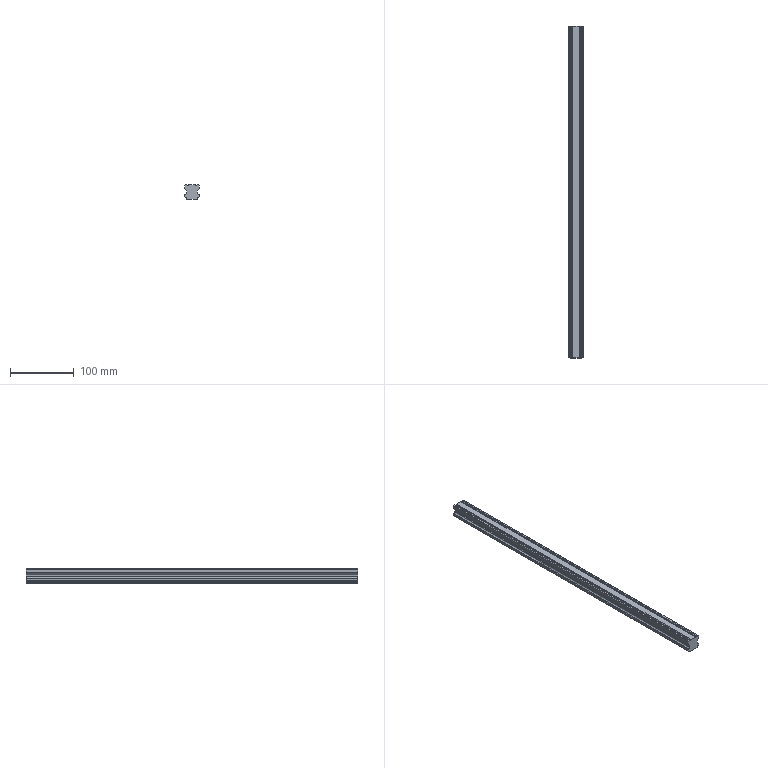Component | SolidWorks | GuideRailHGH25-2-1 | 1 solid | 34 faces | box 23 x 520 x 22 mm | volume 228766 mm3 | plane 30 | cylinder 4 | commonest cylinder face diameters 4.6 x4
build123d program:
from build123d import *

# Parameters (mm, degrees)
BOSS_EXTRUDE1_DEPTH = 260


with BuildPart() as part:
    # Sketch1 → Boss-Extrude1 (new, symmetric)
    with BuildSketch(Plane.XY):
        with BuildLine():
            Line((-10.5, 0), (-8.214, 0))
            Line((-8.214, 0), (-7.448, 0.7667))
            Line((-7.448, 0.7667), (-5.695, 0.7667))
            Line((-5.695, 0.7667), (-4.929, 0))
            Line((-4.929, 0), (4.929, 0))
            Line((4.929, 0), (5.695, 0.7667))
            Line((5.695, 0.7667), (7.448, 0.7667))
            Line((7.448, 0.7667), (8.214, 0))
            Line((8.214, 0), (10.5, 0))
            Line((10.5, 0), (11.5, 1))
            Line((11.5, 1), (11.5, 5.5))
            Line((11.5, 5.5), (8.05, 8.95))
            Line((8.05, 8.95), (8.05, 11.95))
            Line((8.05, 11.95), (8.699, 12.599))
            ThreePointArc((8.699, 12.599), (9.368, 14.082), (10.851, 14.751))
            Line((10.851, 14.751), (11.5, 15.4))
            Line((11.5, 15.4), (11.5, 18.55))
            Line((11.5, 18.55), (10.851, 19.199))
            ThreePointArc((10.851, 19.199), (9.368, 19.868), (8.699, 21.351))
            Line((8.699, 21.351), (8.05, 22))
            Line((8.05, 22), (-8.05, 22))
            Line((-8.05, 22), (-8.699, 21.351))
            ThreePointArc((-8.699, 21.351), (-9.368, 19.868), (-10.851, 19.199))
            Line((-10.851, 19.199), (-11.5, 18.55))
            Line((-11.5, 18.55), (-11.5, 15.4))
            Line((-11.5, 15.4), (-10.851, 14.751))
            ThreePointArc((-10.851, 14.751), (-9.368, 14.082), (-8.699, 12.599))
            Line((-8.699, 12.599), (-8.05, 11.95))
            Line((-8.05, 11.95), (-8.05, 8.95))
            Line((-8.05, 8.95), (-11.5, 5.5))
            Line((-11.5, 5.5), (-11.5, 1))
            Line((-11.5, 1), (-10.5, 0))
        make_face()
    extrude(amount=BOSS_EXTRUDE1_DEPTH, both=True)


solid = part.part

# Placed as in the assembly
solid = solid.moved(Location((90.729, -43.5, -24.5), (-90, 0, 0)))
STEP:
#1=COLOUR_RGB('',0.7922,0.8196,0.9333);
#2=FILL_AREA_STYLE_COLOUR('',#1);
#3=FILL_AREA_STYLE('',(#2));
#4=SURFACE_STYLE_FILL_AREA(#3);
#5=SURFACE_SIDE_STYLE('',(#4));
#6=SURFACE_STYLE_USAGE(.BOTH.,#5);
#7=PRESENTATION_STYLE_ASSIGNMENT((#6));
#8=CARTESIAN_POINT('',(3.915,-11.949,-1.805));
#9=VERTEX_POINT('',#8);
#10=CARTESIAN_POINT('',(3.889,-11.949,-1.831));
#11=VERTEX_POINT('',#10);
#12=CARTESIAN_POINT('',(3.915,-11.949,-1.805));
#13=DIRECTION('',(-0.7071,0.,-0.7071));
#14=VECTOR('',#13,39.37);
#15=LINE('',#12,#14);
#16=EDGE_CURVE('',#9,#11,#15,.T.);
#17=ORIENTED_EDGE('',*,*,#16,.T.);
#18=CARTESIAN_POINT('',(3.889,8.524,-1.831));
#19=VERTEX_POINT('',#18);
#20=CARTESIAN_POINT('',(3.889,8.524,-1.831));
#21=DIRECTION('',(0.,-1.,-0.));
#22=VECTOR('',#21,39.37);
#23=LINE('',#20,#22);
#24=EDGE_CURVE('',#19,#11,#23,.T.);
#25=ORIENTED_EDGE('',*,*,#24,.F.);
#26=CARTESIAN_POINT('',(3.915,8.524,-1.805));
#27=VERTEX_POINT('',#26);
#28=CARTESIAN_POINT('',(3.915,8.524,-1.805));
#29=DIRECTION('',(-0.7071,0.,-0.7071));
#30=VECTOR('',#29,39.37);
#31=LINE('',#28,#30);
#32=EDGE_CURVE('',#27,#19,#31,.T.);
#33=ORIENTED_EDGE('',*,*,#32,.F.);
#34=CARTESIAN_POINT('',(3.915,8.524,-1.805));
#35=DIRECTION('',(0.,-1.,-0.));
#36=VECTOR('',#35,39.37);
#37=LINE('',#34,#36);
#38=EDGE_CURVE('',#27,#9,#37,.T.);
#39=ORIENTED_EDGE('',*,*,#38,.T.);
#40=EDGE_LOOP('',(#17,#25,#33,#39));
#41=FACE_OUTER_BOUND('',#40,.T.);
#42=CARTESIAN_POINT('',(3.915,8.524,-1.805));
#43=DIRECTION('',(-0.7071,-0.,0.7071));
#44=DIRECTION('',(0.7071,-0.,0.7071));
#45=AXIS2_PLACEMENT_3D('',#42,#43,#44);
#46=PLANE('',#45);
#47=ADVANCED_FACE('',(#41),#46,.F.);
#48=CARTESIAN_POINT('',(3.255,-11.949,-1.831));
#49=VERTEX_POINT('',#48);
#50=CARTESIAN_POINT('',(3.889,-11.949,-1.831));
#51=DIRECTION('',(-1.,-0.,-0.));
#52=VECTOR('',#51,39.37);
#53=LINE('',#50,#52);
#54=EDGE_CURVE('',#11,#49,#53,.T.);
#55=ORIENTED_EDGE('',*,*,#54,.T.);
#56=CARTESIAN_POINT('',(3.255,8.524,-1.831));
#57=VERTEX_POINT('',#56);
#58=CARTESIAN_POINT('',(3.255,8.524,-1.831));
#59=DIRECTION('',(0.,-1.,-0.));
#60=VECTOR('',#59,39.37);
#61=LINE('',#58,#60);
#62=EDGE_CURVE('',#57,#49,#61,.T.);
#63=ORIENTED_EDGE('',*,*,#62,.F.);
#64=CARTESIAN_POINT('',(3.889,8.524,-1.831));
#65=DIRECTION('',(-1.,-0.,-0.));
#66=VECTOR('',#65,39.37);
#67=LINE('',#64,#66);
#68=EDGE_CURVE('',#19,#57,#67,.T.);
#69=ORIENTED_EDGE('',*,*,#68,.F.);
#70=ORIENTED_EDGE('',*,*,#24,.T.);
#71=EDGE_LOOP('',(#55,#63,#69,#70));
#72=FACE_OUTER_BOUND('',#71,.T.);
#73=CARTESIAN_POINT('',(3.889,8.524,-1.831));
#74=DIRECTION('',(-0.,-0.,1.));
#75=DIRECTION('',(1.,0.,0.));
#76=AXIS2_PLACEMENT_3D('',#73,#74,#75);
#77=PLANE('',#76);
#78=ADVANCED_FACE('',(#72),#77,.F.);
#79=CARTESIAN_POINT('',(3.23,-11.949,-1.805));
#80=VERTEX_POINT('',#79);
#81=CARTESIAN_POINT('',(3.255,-11.949,-1.831));
#82=DIRECTION('',(-0.7071,-0.,0.7071));
#83=VECTOR('',#82,39.37);
#84=LINE('',#81,#83);
#85=EDGE_CURVE('',#49,#80,#84,.T.);
#86=ORIENTED_EDGE('',*,*,#85,.T.);
#87=CARTESIAN_POINT('',(3.23,8.524,-1.805));
#88=VERTEX_POINT('',#87);
#89=CARTESIAN_POINT('',(3.23,8.524,-1.805));
#90=DIRECTION('',(0.,-1.,-0.));
#91=VECTOR('',#90,39.37);
#92=LINE('',#89,#91);
#93=EDGE_CURVE('',#88,#80,#92,.T.);
#94=ORIENTED_EDGE('',*,*,#93,.F.);
#95=CARTESIAN_POINT('',(3.255,8.524,-1.831));
#96=DIRECTION('',(-0.7071,-0.,0.7071));
#97=VECTOR('',#96,39.37);
#98=LINE('',#95,#97);
#99=EDGE_CURVE('',#57,#88,#98,.T.);
#100=ORIENTED_EDGE('',*,*,#99,.F.);
#101=ORIENTED_EDGE('',*,*,#62,.T.);
#102=EDGE_LOOP('',(#86,#94,#100,#101));
#103=FACE_OUTER_BOUND('',#102,.T.);
#104=CARTESIAN_POINT('',(3.255,8.524,-1.831));
#105=DIRECTION('',(0.7071,-0.,0.7071));
#106=DIRECTION('',(0.7071,0.,-0.7071));
#107=AXIS2_PLACEMENT_3D('',#104,#105,#106);
#108=PLANE('',#107);
#109=ADVANCED_FACE('',(#103),#108,.F.);
#110=CARTESIAN_POINT('',(3.145,-11.949,-1.72));
#111=VERTEX_POINT('',#110);
#112=CARTESIAN_POINT('',(3.139,-11.949,-1.811));
#113=DIRECTION('',(-0.,1.,0.));
#114=DIRECTION('',(1.,0.,0.));
#115=AXIS2_PLACEMENT_3D('',#112,#113,#114);
#116=CIRCLE('',#115,0.09055);
#117=EDGE_CURVE('',#111,#80,#116,.T.);
#118=ORIENTED_EDGE('',*,*,#117,.F.);
#119=CARTESIAN_POINT('',(3.145,8.524,-1.72));
#120=VERTEX_POINT('',#119);
#121=CARTESIAN_POINT('',(3.145,8.524,-1.72));
#122=DIRECTION('',(0.,-1.,-0.));
#123=VECTOR('',#122,39.37);
#124=LINE('',#121,#123);
#125=EDGE_CURVE('',#120,#111,#124,.T.);
#126=ORIENTED_EDGE('',*,*,#125,.F.);
#127=CARTESIAN_POINT('',(3.139,8.524,-1.811));
#128=DIRECTION('',(-0.,1.,0.));
#129=DIRECTION('',(1.,0.,0.));
#130=AXIS2_PLACEMENT_3D('',#127,#128,#129);
#131=CIRCLE('',#130,0.09055);
#132=EDGE_CURVE('',#120,#88,#131,.T.);
#133=ORIENTED_EDGE('',*,*,#132,.T.);
#134=ORIENTED_EDGE('',*,*,#93,.T.);
#135=EDGE_LOOP('',(#118,#126,#133,#134));
#136=FACE_OUTER_BOUND('',#135,.T.);
#137=CARTESIAN_POINT('',(3.139,8.524,-1.811));
#138=DIRECTION('',(0.,-1.,-0.));
#139=DIRECTION('',(-1.,0.,-0.));
#140=AXIS2_PLACEMENT_3D('',#137,#138,#139);
#141=CYLINDRICAL_SURFACE('',#140,0.09055);
#142=ADVANCED_FACE('',(#136),#141,.F.);
#143=CARTESIAN_POINT('',(3.119,-11.949,-1.695));
#144=VERTEX_POINT('',#143);
#145=CARTESIAN_POINT('',(3.145,-11.949,-1.72));
#146=DIRECTION('',(-0.7071,-0.,0.7071));
#147=VECTOR('',#146,39.37);
#148=LINE('',#145,#147);
#149=EDGE_CURVE('',#111,#144,#148,.T.);
#150=ORIENTED_EDGE('',*,*,#149,.T.);
#151=CARTESIAN_POINT('',(3.119,8.524,-1.695));
#152=VERTEX_POINT('',#151);
#153=CARTESIAN_POINT('',(3.119,8.524,-1.695));
#154=DIRECTION('',(0.,-1.,-0.));
#155=VECTOR('',#154,39.37);
#156=LINE('',#153,#155);
#157=EDGE_CURVE('',#152,#144,#156,.T.);
#158=ORIENTED_EDGE('',*,*,#157,.F.);
#159=CARTESIAN_POINT('',(3.145,8.524,-1.72));
#160=DIRECTION('',(-0.7071,-0.,0.7071));
#161=VECTOR('',#160,39.37);
#162=LINE('',#159,#161);
#163=EDGE_CURVE('',#120,#152,#162,.T.);
#164=ORIENTED_EDGE('',*,*,#163,.F.);
#165=ORIENTED_EDGE('',*,*,#125,.T.);
#166=EDGE_LOOP('',(#150,#158,#164,#165));
#167=FACE_OUTER_BOUND('',#166,.T.);
#168=CARTESIAN_POINT('',(3.145,8.524,-1.72));
#169=DIRECTION('',(0.7071,-0.,0.7071));
#170=DIRECTION('',(0.7071,0.,-0.7071));
#171=AXIS2_PLACEMENT_3D('',#168,#169,#170);
#172=PLANE('',#171);
#173=ADVANCED_FACE('',(#167),#172,.F.);
#174=CARTESIAN_POINT('',(3.119,-11.949,-1.571));
#175=VERTEX_POINT('',#174);
#176=CARTESIAN_POINT('',(3.119,-11.949,-1.695));
#177=DIRECTION('',(-0.,-0.,1.));
#178=VECTOR('',#177,39.37);
#179=LINE('',#176,#178);
#180=EDGE_CURVE('',#144,#175,#179,.T.);
#181=ORIENTED_EDGE('',*,*,#180,.T.);
#182=CARTESIAN_POINT('',(3.119,8.524,-1.571));
#183=VERTEX_POINT('',#182);
#184=CARTESIAN_POINT('',(3.119,8.524,-1.571));
#185=DIRECTION('',(0.,-1.,-0.));
#186=VECTOR('',#185,39.37);
#187=LINE('',#184,#186);
#188=EDGE_CURVE('',#183,#175,#187,.T.);
#189=ORIENTED_EDGE('',*,*,#188,.F.);
#190=CARTESIAN_POINT('',(3.119,8.524,-1.695));
#191=DIRECTION('',(-0.,-0.,1.));
#192=VECTOR('',#191,39.37);
#193=LINE('',#190,#192);
#194=EDGE_CURVE('',#152,#183,#193,.T.);
#195=ORIENTED_EDGE('',*,*,#194,.F.);
#196=ORIENTED_EDGE('',*,*,#157,.T.);
#197=EDGE_LOOP('',(#181,#189,#195,#196));
#198=FACE_OUTER_BOUND('',#197,.T.);
#199=CARTESIAN_POINT('',(3.119,8.524,-1.695));
#200=DIRECTION('',(1.,0.,0.));
#201=DIRECTION('',(0.,-1.,-0.));
#202=AXIS2_PLACEMENT_3D('',#199,#200,#201);
#203=PLANE('',#202);
#204=ADVANCED_FACE('',(#198),#203,.F.);
#205=CARTESIAN_POINT('',(3.145,-11.949,-1.545));
#206=VERTEX_POINT('',#205);
#207=CARTESIAN_POINT('',(3.119,-11.949,-1.571));
#208=DIRECTION('',(0.7071,-0.,0.7071));
#209=VECTOR('',#208,39.37);
#210=LINE('',#207,#209);
#211=EDGE_CURVE('',#175,#206,#210,.T.);
#212=ORIENTED_EDGE('',*,*,#211,.T.);
#213=CARTESIAN_POINT('',(3.145,8.524,-1.545));
#214=VERTEX_POINT('',#213);
#215=CARTESIAN_POINT('',(3.145,8.524,-1.545));
#216=DIRECTION('',(0.,-1.,-0.));
#217=VECTOR('',#216,39.37);
#218=LINE('',#215,#217);
#219=EDGE_CURVE('',#214,#206,#218,.T.);
#220=ORIENTED_EDGE('',*,*,#219,.F.);
#221=CARTESIAN_POINT('',(3.119,8.524,-1.571));
#222=DIRECTION('',(0.7071,-0.,0.7071));
#223=VECTOR('',#222,39.37);
#224=LINE('',#221,#223);
#225=EDGE_CURVE('',#183,#214,#224,.T.);
#226=ORIENTED_EDGE('',*,*,#225,.F.);
#227=ORIENTED_EDGE('',*,*,#188,.T.);
#228=EDGE_LOOP('',(#212,#220,#226,#227));
#229=FACE_OUTER_BOUND('',#228,.T.);
#230=CARTESIAN_POINT('',(3.119,8.524,-1.571));
#231=DIRECTION('',(0.7071,0.,-0.7071));
#232=DIRECTION('',(-0.7071,0.,-0.7071));
#233=AXIS2_PLACEMENT_3D('',#230,#231,#232);
#234=PLANE('',#233);
#235=ADVANCED_FACE('',(#229),#234,.F.);
#236=CARTESIAN_POINT('',(3.23,-11.949,-1.461));
#237=VERTEX_POINT('',#236);
#238=CARTESIAN_POINT('',(3.139,-11.949,-1.455));
#239=DIRECTION('',(-0.,1.,0.));
#240=DIRECTION('',(1.,0.,0.));
#241=AXIS2_PLACEMENT_3D('',#238,#239,#240);
#242=CIRCLE('',#241,0.09055);
#243=EDGE_CURVE('',#237,#206,#242,.T.);
#244=ORIENTED_EDGE('',*,*,#243,.F.);
#245=CARTESIAN_POINT('',(3.23,8.524,-1.461));
#246=VERTEX_POINT('',#245);
#247=CARTESIAN_POINT('',(3.23,8.524,-1.461));
#248=DIRECTION('',(0.,-1.,-0.));
#249=VECTOR('',#248,39.37);
#250=LINE('',#247,#249);
#251=EDGE_CURVE('',#246,#237,#250,.T.);
#252=ORIENTED_EDGE('',*,*,#251,.F.);
#253=CARTESIAN_POINT('',(3.139,8.524,-1.455));
#254=DIRECTION('',(-0.,1.,0.));
#255=DIRECTION('',(1.,0.,0.));
#256=AXIS2_PLACEMENT_3D('',#253,#254,#255);
#257=CIRCLE('',#256,0.09055);
#258=EDGE_CURVE('',#246,#214,#257,.T.);
#259=ORIENTED_EDGE('',*,*,#258,.T.);
#260=ORIENTED_EDGE('',*,*,#219,.T.);
#261=EDGE_LOOP('',(#244,#252,#259,#260));
#262=FACE_OUTER_BOUND('',#261,.T.);
#263=CARTESIAN_POINT('',(3.139,8.524,-1.455));
#264=DIRECTION('',(0.,-1.,-0.));
#265=DIRECTION('',(-1.,0.,-0.));
#266=AXIS2_PLACEMENT_3D('',#263,#264,#265);
#267=CYLINDRICAL_SURFACE('',#266,0.09055);
#268=ADVANCED_FACE('',(#262),#267,.F.);
#269=CARTESIAN_POINT('',(3.255,-11.949,-1.435));
#270=VERTEX_POINT('',#269);
#271=CARTESIAN_POINT('',(3.23,-11.949,-1.461));
#272=DIRECTION('',(0.7071,-0.,0.7071));
#273=VECTOR('',#272,39.37);
#274=LINE('',#271,#273);
#275=EDGE_CURVE('',#237,#270,#274,.T.);
#276=ORIENTED_EDGE('',*,*,#275,.T.);
#277=CARTESIAN_POINT('',(3.255,8.524,-1.435));
#278=VERTEX_POINT('',#277);
#279=CARTESIAN_POINT('',(3.255,8.524,-1.435));
#280=DIRECTION('',(0.,-1.,-0.));
#281=VECTOR('',#280,39.37);
#282=LINE('',#279,#281);
#283=EDGE_CURVE('',#278,#270,#282,.T.);
#284=ORIENTED_EDGE('',*,*,#283,.F.);
#285=CARTESIAN_POINT('',(3.23,8.524,-1.461));
#286=DIRECTION('',(0.7071,-0.,0.7071));
#287=VECTOR('',#286,39.37);
#288=LINE('',#285,#287);
#289=EDGE_CURVE('',#246,#278,#288,.T.);
#290=ORIENTED_EDGE('',*,*,#289,.F.);
#291=ORIENTED_EDGE('',*,*,#251,.T.);
#292=EDGE_LOOP('',(#276,#284,#290,#291));
#293=FACE_OUTER_BOUND('',#292,.T.);
#294=CARTESIAN_POINT('',(3.23,8.524,-1.461));
#295=DIRECTION('',(0.7071,0.,-0.7071));
#296=DIRECTION('',(-0.7071,0.,-0.7071));
#297=AXIS2_PLACEMENT_3D('',#294,#295,#296);
#298=PLANE('',#297);
#299=ADVANCED_FACE('',(#293),#298,.F.);
#300=CARTESIAN_POINT('',(3.255,-11.949,-1.317));
#301=VERTEX_POINT('',#300);
#302=CARTESIAN_POINT('',(3.255,-11.949,-1.435));
#303=DIRECTION('',(-0.,-0.,1.));
#304=VECTOR('',#303,39.37);
#305=LINE('',#302,#304);
#306=EDGE_CURVE('',#270,#301,#305,.T.);
#307=ORIENTED_EDGE('',*,*,#306,.T.);
#308=CARTESIAN_POINT('',(3.255,8.524,-1.317));
#309=VERTEX_POINT('',#308);
#310=CARTESIAN_POINT('',(3.255,8.524,-1.317));
#311=DIRECTION('',(0.,-1.,-0.));
#312=VECTOR('',#311,39.37);
#313=LINE('',#310,#312);
#314=EDGE_CURVE('',#309,#301,#313,.T.);
#315=ORIENTED_EDGE('',*,*,#314,.F.);
#316=CARTESIAN_POINT('',(3.255,8.524,-1.435));
#317=DIRECTION('',(-0.,-0.,1.));
#318=VECTOR('',#317,39.37);
#319=LINE('',#316,#318);
#320=EDGE_CURVE('',#278,#309,#319,.T.);
#321=ORIENTED_EDGE('',*,*,#320,.F.);
#322=ORIENTED_EDGE('',*,*,#283,.T.);
#323=EDGE_LOOP('',(#307,#315,#321,#322));
#324=FACE_OUTER_BOUND('',#323,.T.);
#325=CARTESIAN_POINT('',(3.255,8.524,-1.435));
#326=DIRECTION('',(1.,0.,0.));
#327=DIRECTION('',(0.,0.,-1.));
#328=AXIS2_PLACEMENT_3D('',#325,#326,#327);
#329=PLANE('',#328);
#330=ADVANCED_FACE('',(#324),#329,.F.);
#331=CARTESIAN_POINT('',(3.119,-11.949,-1.181));
#332=VERTEX_POINT('',#331);
#333=CARTESIAN_POINT('',(3.255,-11.949,-1.317));
#334=DIRECTION('',(-0.7071,-0.,0.7071));
#335=VECTOR('',#334,39.37);
#336=LINE('',#333,#335);
#337=EDGE_CURVE('',#301,#332,#336,.T.);
#338=ORIENTED_EDGE('',*,*,#337,.T.);
#339=CARTESIAN_POINT('',(3.119,8.524,-1.181));
#340=VERTEX_POINT('',#339);
#341=CARTESIAN_POINT('',(3.119,8.524,-1.181));
#342=DIRECTION('',(0.,-1.,-0.));
#343=VECTOR('',#342,39.37);
#344=LINE('',#341,#343);
#345=EDGE_CURVE('',#340,#332,#344,.T.);
#346=ORIENTED_EDGE('',*,*,#345,.F.);
#347=CARTESIAN_POINT('',(3.255,8.524,-1.317));
#348=DIRECTION('',(-0.7071,-0.,0.7071));
#349=VECTOR('',#348,39.37);
#350=LINE('',#347,#349);
#351=EDGE_CURVE('',#309,#340,#350,.T.);
#352=ORIENTED_EDGE('',*,*,#351,.F.);
#353=ORIENTED_EDGE('',*,*,#314,.T.);
#354=EDGE_LOOP('',(#338,#346,#352,#353));
#355=FACE_OUTER_BOUND('',#354,.T.);
#356=CARTESIAN_POINT('',(3.255,8.524,-1.317));
#357=DIRECTION('',(0.7071,-0.,0.7071));
#358=DIRECTION('',(0.7071,0.,-0.7071));
#359=AXIS2_PLACEMENT_3D('',#356,#357,#358);
#360=PLANE('',#359);
#361=ADVANCED_FACE('',(#355),#360,.F.);
#362=CARTESIAN_POINT('',(3.119,-11.949,-1.004));
#363=VERTEX_POINT('',#362);
#364=CARTESIAN_POINT('',(3.119,-11.949,-1.181));
#365=DIRECTION('',(-0.,-0.,1.));
#366=VECTOR('',#365,39.37);
#367=LINE('',#364,#366);
#368=EDGE_CURVE('',#332,#363,#367,.T.);
#369=ORIENTED_EDGE('',*,*,#368,.T.);
#370=CARTESIAN_POINT('',(3.119,8.524,-1.004));
#371=VERTEX_POINT('',#370);
#372=CARTESIAN_POINT('',(3.119,8.524,-1.004));
#373=DIRECTION('',(0.,-1.,-0.));
#374=VECTOR('',#373,39.37);
#375=LINE('',#372,#374);
#376=EDGE_CURVE('',#371,#363,#375,.T.);
#377=ORIENTED_EDGE('',*,*,#376,.F.);
#378=CARTESIAN_POINT('',(3.119,8.524,-1.181));
#379=DIRECTION('',(-0.,-0.,1.));
#380=VECTOR('',#379,39.37);
#381=LINE('',#378,#380);
#382=EDGE_CURVE('',#340,#371,#381,.T.);
#383=ORIENTED_EDGE('',*,*,#382,.F.);
#384=ORIENTED_EDGE('',*,*,#345,.T.);
#385=EDGE_LOOP('',(#369,#377,#383,#384));
#386=FACE_OUTER_BOUND('',#385,.T.);
#387=CARTESIAN_POINT('',(3.119,8.524,-1.181));
#388=DIRECTION('',(1.,0.,0.));
#389=DIRECTION('',(0.,-1.,-0.));
#390=AXIS2_PLACEMENT_3D('',#387,#388,#389);
#391=PLANE('',#390);
#392=ADVANCED_FACE('',(#386),#391,.F.);
#393=CARTESIAN_POINT('',(3.159,-11.949,-0.9646));
#394=VERTEX_POINT('',#393);
#395=CARTESIAN_POINT('',(3.119,-11.949,-1.004));
#396=DIRECTION('',(0.7071,-0.,0.7071));
#397=VECTOR('',#396,39.37);
#398=LINE('',#395,#397);
#399=EDGE_CURVE('',#363,#394,#398,.T.);
#400=ORIENTED_EDGE('',*,*,#399,.T.);
#401=CARTESIAN_POINT('',(3.159,8.524,-0.9646));
#402=VERTEX_POINT('',#401);
#403=CARTESIAN_POINT('',(3.159,8.524,-0.9646));
#404=DIRECTION('',(0.,-1.,-0.));
#405=VECTOR('',#404,39.37);
#406=LINE('',#403,#405);
#407=EDGE_CURVE('',#402,#394,#406,.T.);
#408=ORIENTED_EDGE('',*,*,#407,.F.);
#409=CARTESIAN_POINT('',(3.119,8.524,-1.004));
#410=DIRECTION('',(0.7071,-0.,0.7071));
#411=VECTOR('',#410,39.37);
#412=LINE('',#409,#411);
#413=EDGE_CURVE('',#371,#402,#412,.T.);
#414=ORIENTED_EDGE('',*,*,#413,.F.);
#415=ORIENTED_EDGE('',*,*,#376,.T.);
#416=EDGE_LOOP('',(#400,#408,#414,#415));
#417=FACE_OUTER_BOUND('',#416,.T.);
#418=CARTESIAN_POINT('',(3.119,8.524,-1.004));
#419=DIRECTION('',(0.7071,0.,-0.7071));
#420=DIRECTION('',(-0.7071,0.,-0.7071));
#421=AXIS2_PLACEMENT_3D('',#418,#419,#420);
#422=PLANE('',#421);
#423=ADVANCED_FACE('',(#417),#422,.F.);
#424=CARTESIAN_POINT('',(3.249,-11.949,-0.9646));
#425=VERTEX_POINT('',#424);
#426=CARTESIAN_POINT('',(3.159,-11.949,-0.9646));
#427=DIRECTION('',(1.,0.,0.));
#428=VECTOR('',#427,39.37);
#429=LINE('',#426,#428);
#430=EDGE_CURVE('',#394,#425,#429,.T.);
#431=ORIENTED_EDGE('',*,*,#430,.T.);
#432=CARTESIAN_POINT('',(3.249,8.524,-0.9646));
#433=VERTEX_POINT('',#432);
#434=CARTESIAN_POINT('',(3.249,8.524,-0.9646));
#435=DIRECTION('',(0.,-1.,-0.));
#436=VECTOR('',#435,39.37);
#437=LINE('',#434,#436);
#438=EDGE_CURVE('',#433,#425,#437,.T.);
#439=ORIENTED_EDGE('',*,*,#438,.F.);
#440=CARTESIAN_POINT('',(3.159,8.524,-0.9646));
#441=DIRECTION('',(1.,0.,0.));
#442=VECTOR('',#441,39.37);
#443=LINE('',#440,#442);
#444=EDGE_CURVE('',#402,#433,#443,.T.);
#445=ORIENTED_EDGE('',*,*,#444,.F.);
#446=ORIENTED_EDGE('',*,*,#407,.T.);
#447=EDGE_LOOP('',(#431,#439,#445,#446));
#448=FACE_OUTER_BOUND('',#447,.T.);
#449=CARTESIAN_POINT('',(3.159,8.524,-0.9646));
#450=DIRECTION('',(0.,0.,-1.));
#451=DIRECTION('',(-1.,-0.,-0.));
#452=AXIS2_PLACEMENT_3D('',#449,#450,#451);
#453=PLANE('',#452);
#454=ADVANCED_FACE('',(#448),#453,.F.);
#455=CARTESIAN_POINT('',(3.279,-11.949,-0.9948));
#456=VERTEX_POINT('',#455);
#457=CARTESIAN_POINT('',(3.249,-11.949,-0.9646));
#458=DIRECTION('',(0.7071,0.,-0.7071));
#459=VECTOR('',#458,39.37);
#460=LINE('',#457,#459);
#461=EDGE_CURVE('',#425,#456,#460,.T.);
#462=ORIENTED_EDGE('',*,*,#461,.T.);
#463=CARTESIAN_POINT('',(3.279,8.524,-0.9948));
#464=VERTEX_POINT('',#463);
#465=CARTESIAN_POINT('',(3.279,8.524,-0.9948));
#466=DIRECTION('',(0.,-1.,-0.));
#467=VECTOR('',#466,39.37);
#468=LINE('',#465,#467);
#469=EDGE_CURVE('',#464,#456,#468,.T.);
#470=ORIENTED_EDGE('',*,*,#469,.F.);
#471=CARTESIAN_POINT('',(3.249,8.524,-0.9646));
#472=DIRECTION('',(0.7071,0.,-0.7071));
#473=VECTOR('',#472,39.37);
#474=LINE('',#471,#473);
#475=EDGE_CURVE('',#433,#464,#474,.T.);
#476=ORIENTED_EDGE('',*,*,#475,.F.);
#477=ORIENTED_EDGE('',*,*,#438,.T.);
#478=EDGE_LOOP('',(#462,#470,#476,#477));
#479=FACE_OUTER_BOUND('',#478,.T.);
#480=CARTESIAN_POINT('',(3.249,8.524,-0.9646));
#481=DIRECTION('',(-0.7071,0.,-0.7071));
#482=DIRECTION('',(-0.7071,-0.,0.7071));
#483=AXIS2_PLACEMENT_3D('',#480,#481,#482);
#484=PLANE('',#483);
#485=ADVANCED_FACE('',(#479),#484,.F.);
#486=CARTESIAN_POINT('',(3.348,-11.949,-0.9948));
#487=VERTEX_POINT('',#486);
#488=CARTESIAN_POINT('',(3.279,-11.949,-0.9948));
#489=DIRECTION('',(1.,0.,-0.));
#490=VECTOR('',#489,39.37);
#491=LINE('',#488,#490);
#492=EDGE_CURVE('',#456,#487,#491,.T.);
#493=ORIENTED_EDGE('',*,*,#492,.T.);
#494=CARTESIAN_POINT('',(3.348,8.524,-0.9948));
#495=VERTEX_POINT('',#494);
#496=CARTESIAN_POINT('',(3.348,8.524,-0.9948));
#497=DIRECTION('',(0.,-1.,-0.));
#498=VECTOR('',#497,39.37);
#499=LINE('',#496,#498);
#500=EDGE_CURVE('',#495,#487,#499,.T.);
#501=ORIENTED_EDGE('',*,*,#500,.F.);
#502=CARTESIAN_POINT('',(3.279,8.524,-0.9948));
#503=DIRECTION('',(1.,0.,-0.));
#504=VECTOR('',#503,39.37);
#505=LINE('',#502,#504);
#506=EDGE_CURVE('',#464,#495,#505,.T.);
#507=ORIENTED_EDGE('',*,*,#506,.F.);
#508=ORIENTED_EDGE('',*,*,#469,.T.);
#509=EDGE_LOOP('',(#493,#501,#507,#508));
#510=FACE_OUTER_BOUND('',#509,.T.);
#511=CARTESIAN_POINT('',(3.279,8.524,-0.9948));
#512=DIRECTION('',(-0.,0.,-1.));
#513=DIRECTION('',(-1.,-0.,0.));
#514=AXIS2_PLACEMENT_3D('',#511,#512,#513);
#515=PLANE('',#514);
#516=ADVANCED_FACE('',(#510),#515,.F.);
#517=CARTESIAN_POINT('',(3.378,-11.949,-0.9646));
#518=VERTEX_POINT('',#517);
#519=CARTESIAN_POINT('',(3.348,-11.949,-0.9948));
#520=DIRECTION('',(0.7071,-0.,0.7071));
#521=VECTOR('',#520,39.37);
#522=LINE('',#519,#521);
#523=EDGE_CURVE('',#487,#518,#522,.T.);
#524=ORIENTED_EDGE('',*,*,#523,.T.);
#525=CARTESIAN_POINT('',(3.378,8.524,-0.9646));
#526=VERTEX_POINT('',#525);
#527=CARTESIAN_POINT('',(3.378,8.524,-0.9646));
#528=DIRECTION('',(0.,-1.,-0.));
#529=VECTOR('',#528,39.37);
#530=LINE('',#527,#529);
#531=EDGE_CURVE('',#526,#518,#530,.T.);
#532=ORIENTED_EDGE('',*,*,#531,.F.);
#533=CARTESIAN_POINT('',(3.348,8.524,-0.9948));
#534=DIRECTION('',(0.7071,-0.,0.7071));
#535=VECTOR('',#534,39.37);
#536=LINE('',#533,#535);
#537=EDGE_CURVE('',#495,#526,#536,.T.);
#538=ORIENTED_EDGE('',*,*,#537,.F.);
#539=ORIENTED_EDGE('',*,*,#500,.T.);
#540=EDGE_LOOP('',(#524,#532,#538,#539));
#541=FACE_OUTER_BOUND('',#540,.T.);
#542=CARTESIAN_POINT('',(3.348,8.524,-0.9948));
#543=DIRECTION('',(0.7071,0.,-0.7071));
#544=DIRECTION('',(-0.7071,0.,-0.7071));
#545=AXIS2_PLACEMENT_3D('',#542,#543,#544);
#546=PLANE('',#545);
#547=ADVANCED_FACE('',(#541),#546,.F.);
#548=CARTESIAN_POINT('',(3.766,-11.949,-0.9646));
#549=VERTEX_POINT('',#548);
#550=CARTESIAN_POINT('',(3.378,-11.949,-0.9646));
#551=DIRECTION('',(1.,0.,0.));
#552=VECTOR('',#551,39.37);
#553=LINE('',#550,#552);
#554=EDGE_CURVE('',#518,#549,#553,.T.);
#555=ORIENTED_EDGE('',*,*,#554,.T.);
#556=CARTESIAN_POINT('',(3.766,8.524,-0.9646));
#557=VERTEX_POINT('',#556);
#558=CARTESIAN_POINT('',(3.766,8.524,-0.9646));
#559=DIRECTION('',(0.,-1.,-0.));
#560=VECTOR('',#559,39.37);
#561=LINE('',#558,#560);
#562=EDGE_CURVE('',#557,#549,#561,.T.);
#563=ORIENTED_EDGE('',*,*,#562,.F.);
#564=CARTESIAN_POINT('',(3.378,8.524,-0.9646));
#565=DIRECTION('',(1.,0.,0.));
#566=VECTOR('',#565,39.37);
#567=LINE('',#564,#566);
#568=EDGE_CURVE('',#526,#557,#567,.T.);
#569=ORIENTED_EDGE('',*,*,#568,.F.);
#570=ORIENTED_EDGE('',*,*,#531,.T.);
#571=EDGE_LOOP('',(#555,#563,#569,#570));
#572=FACE_OUTER_BOUND('',#571,.T.);
#573=CARTESIAN_POINT('',(3.378,8.524,-0.9646));
#574=DIRECTION('',(0.,0.,-1.));
#575=DIRECTION('',(-1.,-0.,-0.));
#576=AXIS2_PLACEMENT_3D('',#573,#574,#575);
#577=PLANE('',#576);
#578=ADVANCED_FACE('',(#572),#577,.F.);
#579=CARTESIAN_POINT('',(3.796,-11.949,-0.9948));
#580=VERTEX_POINT('',#579);
#581=CARTESIAN_POINT('',(3.766,-11.949,-0.9646));
#582=DIRECTION('',(0.7071,0.,-0.7071));
#583=VECTOR('',#582,39.37);
#584=LINE('',#581,#583);
#585=EDGE_CURVE('',#549,#580,#584,.T.);
#586=ORIENTED_EDGE('',*,*,#585,.T.);
#587=CARTESIAN_POINT('',(3.796,8.524,-0.9948));
#588=VERTEX_POINT('',#587);
#589=CARTESIAN_POINT('',(3.796,8.524,-0.9948));
#590=DIRECTION('',(0.,-1.,-0.));
#591=VECTOR('',#590,39.37);
#592=LINE('',#589,#591);
#593=EDGE_CURVE('',#588,#580,#592,.T.);
#594=ORIENTED_EDGE('',*,*,#593,.F.);
#595=CARTESIAN_POINT('',(3.766,8.524,-0.9646));
#596=DIRECTION('',(0.7071,0.,-0.7071));
#597=VECTOR('',#596,39.37);
#598=LINE('',#595,#597);
#599=EDGE_CURVE('',#557,#588,#598,.T.);
#600=ORIENTED_EDGE('',*,*,#599,.F.);
#601=ORIENTED_EDGE('',*,*,#562,.T.);
#602=EDGE_LOOP('',(#586,#594,#600,#601));
#603=FACE_OUTER_BOUND('',#602,.T.);
#604=CARTESIAN_POINT('',(3.766,8.524,-0.9646));
#605=DIRECTION('',(-0.7071,0.,-0.7071));
#606=DIRECTION('',(-0.7071,-0.,0.7071));
#607=AXIS2_PLACEMENT_3D('',#604,#605,#606);
#608=PLANE('',#607);
#609=ADVANCED_FACE('',(#603),#608,.F.);
#610=CARTESIAN_POINT('',(3.865,-11.949,-0.9948));
#611=VERTEX_POINT('',#610);
#612=CARTESIAN_POINT('',(3.796,-11.949,-0.9948));
#613=DIRECTION('',(1.,0.,0.));
#614=VECTOR('',#613,39.37);
#615=LINE('',#612,#614);
#616=EDGE_CURVE('',#580,#611,#615,.T.);
#617=ORIENTED_EDGE('',*,*,#616,.T.);
#618=CARTESIAN_POINT('',(3.865,8.524,-0.9948));
#619=VERTEX_POINT('',#618);
#620=CARTESIAN_POINT('',(3.865,8.524,-0.9948));
#621=DIRECTION('',(0.,-1.,-0.));
#622=VECTOR('',#621,39.37);
#623=LINE('',#620,#622);
#624=EDGE_CURVE('',#619,#611,#623,.T.);
#625=ORIENTED_EDGE('',*,*,#624,.F.);
#626=CARTESIAN_POINT('',(3.796,8.524,-0.9948));
#627=DIRECTION('',(1.,0.,0.));
#628=VECTOR('',#627,39.37);
#629=LINE('',#626,#628);
#630=EDGE_CURVE('',#588,#619,#629,.T.);
#631=ORIENTED_EDGE('',*,*,#630,.F.);
#632=ORIENTED_EDGE('',*,*,#593,.T.);
#633=EDGE_LOOP('',(#617,#625,#631,#632));
#634=FACE_OUTER_BOUND('',#633,.T.);
#635=CARTESIAN_POINT('',(3.796,8.524,-0.9948));
#636=DIRECTION('',(0.,0.,-1.));
#637=DIRECTION('',(-1.,-0.,-0.));
#638=AXIS2_PLACEMENT_3D('',#635,#636,#637);
#639=PLANE('',#638);
#640=ADVANCED_FACE('',(#634),#639,.F.);
#641=CARTESIAN_POINT('',(3.895,-11.949,-0.9646));
#642=VERTEX_POINT('',#641);
#643=CARTESIAN_POINT('',(3.865,-11.949,-0.9948));
#644=DIRECTION('',(0.7071,-0.,0.7071));
#645=VECTOR('',#644,39.37);
#646=LINE('',#643,#645);
#647=EDGE_CURVE('',#611,#642,#646,.T.);
#648=ORIENTED_EDGE('',*,*,#647,.T.);
#649=CARTESIAN_POINT('',(3.895,8.524,-0.9646));
#650=VERTEX_POINT('',#649);
#651=CARTESIAN_POINT('',(3.895,8.524,-0.9646));
#652=DIRECTION('',(0.,-1.,-0.));
#653=VECTOR('',#652,39.37);
#654=LINE('',#651,#653);
#655=EDGE_CURVE('',#650,#642,#654,.T.);
#656=ORIENTED_EDGE('',*,*,#655,.F.);
#657=CARTESIAN_POINT('',(3.865,8.524,-0.9948));
#658=DIRECTION('',(0.7071,-0.,0.7071));
#659=VECTOR('',#658,39.37);
#660=LINE('',#657,#659);
#661=EDGE_CURVE('',#619,#650,#660,.T.);
#662=ORIENTED_EDGE('',*,*,#661,.F.);
#663=ORIENTED_EDGE('',*,*,#624,.T.);
#664=EDGE_LOOP('',(#648,#656,#662,#663));
#665=FACE_OUTER_BOUND('',#664,.T.);
#666=CARTESIAN_POINT('',(3.865,8.524,-0.9948));
#667=DIRECTION('',(0.7071,0.,-0.7071));
#668=DIRECTION('',(-0.7071,0.,-0.7071));
#669=AXIS2_PLACEMENT_3D('',#666,#667,#668);
#670=PLANE('',#669);
#671=ADVANCED_FACE('',(#665),#670,.F.);
#672=CARTESIAN_POINT('',(3.985,-11.949,-0.9646));
#673=VERTEX_POINT('',#672);
#674=CARTESIAN_POINT('',(3.895,-11.949,-0.9646));
#675=DIRECTION('',(1.,0.,0.));
#676=VECTOR('',#675,39.37);
#677=LINE('',#674,#676);
#678=EDGE_CURVE('',#642,#673,#677,.T.);
#679=ORIENTED_EDGE('',*,*,#678,.T.);
#680=CARTESIAN_POINT('',(3.985,8.524,-0.9646));
#681=VERTEX_POINT('',#680);
#682=CARTESIAN_POINT('',(3.985,8.524,-0.9646));
#683=DIRECTION('',(0.,-1.,-0.));
#684=VECTOR('',#683,39.37);
#685=LINE('',#682,#684);
#686=EDGE_CURVE('',#681,#673,#685,.T.);
#687=ORIENTED_EDGE('',*,*,#686,.F.);
#688=CARTESIAN_POINT('',(3.895,8.524,-0.9646));
#689=DIRECTION('',(1.,0.,0.));
#690=VECTOR('',#689,39.37);
#691=LINE('',#688,#690);
#692=EDGE_CURVE('',#650,#681,#691,.T.);
#693=ORIENTED_EDGE('',*,*,#692,.F.);
#694=ORIENTED_EDGE('',*,*,#655,.T.);
#695=EDGE_LOOP('',(#679,#687,#693,#694));
#696=FACE_OUTER_BOUND('',#695,.T.);
#697=CARTESIAN_POINT('',(3.895,8.524,-0.9646));
#698=DIRECTION('',(0.,0.,-1.));
#699=DIRECTION('',(-1.,-0.,-0.));
#700=AXIS2_PLACEMENT_3D('',#697,#698,#699);
#701=PLANE('',#700);
#702=ADVANCED_FACE('',(#696),#701,.F.);
#703=CARTESIAN_POINT('',(4.025,-11.949,-1.004));
#704=VERTEX_POINT('',#703);
#705=CARTESIAN_POINT('',(3.985,-11.949,-0.9646));
#706=DIRECTION('',(0.7071,0.,-0.7071));
#707=VECTOR('',#706,39.37);
#708=LINE('',#705,#707);
#709=EDGE_CURVE('',#673,#704,#708,.T.);
#710=ORIENTED_EDGE('',*,*,#709,.T.);
#711=CARTESIAN_POINT('',(4.025,8.524,-1.004));
#712=VERTEX_POINT('',#711);
#713=CARTESIAN_POINT('',(4.025,8.524,-1.004));
#714=DIRECTION('',(0.,-1.,-0.));
#715=VECTOR('',#714,39.37);
#716=LINE('',#713,#715);
#717=EDGE_CURVE('',#712,#704,#716,.T.);
#718=ORIENTED_EDGE('',*,*,#717,.F.);
#719=CARTESIAN_POINT('',(3.985,8.524,-0.9646));
#720=DIRECTION('',(0.7071,0.,-0.7071));
#721=VECTOR('',#720,39.37);
#722=LINE('',#719,#721);
#723=EDGE_CURVE('',#681,#712,#722,.T.);
#724=ORIENTED_EDGE('',*,*,#723,.F.);
#725=ORIENTED_EDGE('',*,*,#686,.T.);
#726=EDGE_LOOP('',(#710,#718,#724,#725));
#727=FACE_OUTER_BOUND('',#726,.T.);
#728=CARTESIAN_POINT('',(3.985,8.524,-0.9646));
#729=DIRECTION('',(-0.7071,0.,-0.7071));
#730=DIRECTION('',(-0.7071,-0.,0.7071));
#731=AXIS2_PLACEMENT_3D('',#728,#729,#730);
#732=PLANE('',#731);
#733=ADVANCED_FACE('',(#727),#732,.F.);
#734=CARTESIAN_POINT('',(4.025,-11.949,-1.181));
#735=VERTEX_POINT('',#734);
#736=CARTESIAN_POINT('',(4.025,-11.949,-1.004));
#737=DIRECTION('',(0.,0.,-1.));
#738=VECTOR('',#737,39.37);
#739=LINE('',#736,#738);
#740=EDGE_CURVE('',#704,#735,#739,.T.);
#741=ORIENTED_EDGE('',*,*,#740,.T.);
#742=CARTESIAN_POINT('',(4.025,8.524,-1.181));
#743=VERTEX_POINT('',#742);
#744=CARTESIAN_POINT('',(4.025,8.524,-1.181));
#745=DIRECTION('',(0.,-1.,-0.));
#746=VECTOR('',#745,39.37);
#747=LINE('',#744,#746);
#748=EDGE_CURVE('',#743,#735,#747,.T.);
#749=ORIENTED_EDGE('',*,*,#748,.F.);
#750=CARTESIAN_POINT('',(4.025,8.524,-1.004));
#751=DIRECTION('',(0.,0.,-1.));
#752=VECTOR('',#751,39.37);
#753=LINE('',#750,#752);
#754=EDGE_CURVE('',#712,#743,#753,.T.);
#755=ORIENTED_EDGE('',*,*,#754,.F.);
#756=ORIENTED_EDGE('',*,*,#717,.T.);
#757=EDGE_LOOP('',(#741,#749,#755,#756));
#758=FACE_OUTER_BOUND('',#757,.T.);
#759=CARTESIAN_POINT('',(4.025,8.524,-1.004));
#760=DIRECTION('',(-1.,-0.,-0.));
#761=DIRECTION('',(-0.,-0.,1.));
#762=AXIS2_PLACEMENT_3D('',#759,#760,#761);
#763=PLANE('',#762);
#764=ADVANCED_FACE('',(#758),#763,.F.);
#765=CARTESIAN_POINT('',(3.889,-11.949,-1.317));
#766=VERTEX_POINT('',#765);
#767=CARTESIAN_POINT('',(4.025,-11.949,-1.181));
#768=DIRECTION('',(-0.7071,0.,-0.7071));
#769=VECTOR('',#768,39.37);
#770=LINE('',#767,#769);
#771=EDGE_CURVE('',#735,#766,#770,.T.);
#772=ORIENTED_EDGE('',*,*,#771,.T.);
#773=CARTESIAN_POINT('',(3.889,8.524,-1.317));
#774=VERTEX_POINT('',#773);
#775=CARTESIAN_POINT('',(3.889,8.524,-1.317));
#776=DIRECTION('',(0.,-1.,-0.));
#777=VECTOR('',#776,39.37);
#778=LINE('',#775,#777);
#779=EDGE_CURVE('',#774,#766,#778,.T.);
#780=ORIENTED_EDGE('',*,*,#779,.F.);
#781=CARTESIAN_POINT('',(4.025,8.524,-1.181));
#782=DIRECTION('',(-0.7071,0.,-0.7071));
#783=VECTOR('',#782,39.37);
#784=LINE('',#781,#783);
#785=EDGE_CURVE('',#743,#774,#784,.T.);
#786=ORIENTED_EDGE('',*,*,#785,.F.);
#787=ORIENTED_EDGE('',*,*,#748,.T.);
#788=EDGE_LOOP('',(#772,#780,#786,#787));
#789=FACE_OUTER_BOUND('',#788,.T.);
#790=CARTESIAN_POINT('',(4.025,8.524,-1.181));
#791=DIRECTION('',(-0.7071,-0.,0.7071));
#792=DIRECTION('',(0.7071,-0.,0.7071));
#793=AXIS2_PLACEMENT_3D('',#790,#791,#792);
#794=PLANE('',#793);
#795=ADVANCED_FACE('',(#789),#794,.F.);
#796=CARTESIAN_POINT('',(3.889,-11.949,-1.435));
#797=VERTEX_POINT('',#796);
#798=CARTESIAN_POINT('',(3.889,-11.949,-1.317));
#799=DIRECTION('',(0.,0.,-1.));
#800=VECTOR('',#799,39.37);
#801=LINE('',#798,#800);
#802=EDGE_CURVE('',#766,#797,#801,.T.);
#803=ORIENTED_EDGE('',*,*,#802,.T.);
#804=CARTESIAN_POINT('',(3.889,8.524,-1.435));
#805=VERTEX_POINT('',#804);
#806=CARTESIAN_POINT('',(3.889,8.524,-1.435));
#807=DIRECTION('',(0.,-1.,-0.));
#808=VECTOR('',#807,39.37);
#809=LINE('',#806,#808);
#810=EDGE_CURVE('',#805,#797,#809,.T.);
#811=ORIENTED_EDGE('',*,*,#810,.F.);
#812=CARTESIAN_POINT('',(3.889,8.524,-1.317));
#813=DIRECTION('',(0.,0.,-1.));
#814=VECTOR('',#813,39.37);
#815=LINE('',#812,#814);
#816=EDGE_CURVE('',#774,#805,#815,.T.);
#817=ORIENTED_EDGE('',*,*,#816,.F.);
#818=ORIENTED_EDGE('',*,*,#779,.T.);
#819=EDGE_LOOP('',(#803,#811,#817,#818));
#820=FACE_OUTER_BOUND('',#819,.T.);
#821=CARTESIAN_POINT('',(3.889,8.524,-1.317));
#822=DIRECTION('',(-1.,-0.,-0.));
#823=DIRECTION('',(-0.,-0.,1.));
#824=AXIS2_PLACEMENT_3D('',#821,#822,#823);
#825=PLANE('',#824);
#826=ADVANCED_FACE('',(#820),#825,.F.);
#827=CARTESIAN_POINT('',(3.915,-11.949,-1.461));
#828=VERTEX_POINT('',#827);
#829=CARTESIAN_POINT('',(3.889,-11.949,-1.435));
#830=DIRECTION('',(0.7071,0.,-0.7071));
#831=VECTOR('',#830,39.37);
#832=LINE('',#829,#831);
#833=EDGE_CURVE('',#797,#828,#832,.T.);
#834=ORIENTED_EDGE('',*,*,#833,.T.);
#835=CARTESIAN_POINT('',(3.915,8.524,-1.461));
#836=VERTEX_POINT('',#835);
#837=CARTESIAN_POINT('',(3.915,8.524,-1.461));
#838=DIRECTION('',(0.,-1.,-0.));
#839=VECTOR('',#838,39.37);
#840=LINE('',#837,#839);
#841=EDGE_CURVE('',#836,#828,#840,.T.);
#842=ORIENTED_EDGE('',*,*,#841,.F.);
#843=CARTESIAN_POINT('',(3.889,8.524,-1.435));
#844=DIRECTION('',(0.7071,0.,-0.7071));
#845=VECTOR('',#844,39.37);
#846=LINE('',#843,#845);
#847=EDGE_CURVE('',#805,#836,#846,.T.);
#848=ORIENTED_EDGE('',*,*,#847,.F.);
#849=ORIENTED_EDGE('',*,*,#810,.T.);
#850=EDGE_LOOP('',(#834,#842,#848,#849));
#851=FACE_OUTER_BOUND('',#850,.T.);
#852=CARTESIAN_POINT('',(3.889,8.524,-1.435));
#853=DIRECTION('',(-0.7071,0.,-0.7071));
#854=DIRECTION('',(-0.7071,-0.,0.7071));
#855=AXIS2_PLACEMENT_3D('',#852,#853,#854);
#856=PLANE('',#855);
#857=ADVANCED_FACE('',(#851),#856,.F.);
#858=CARTESIAN_POINT('',(3.999,-11.949,-1.545));
#859=VERTEX_POINT('',#858);
#860=CARTESIAN_POINT('',(4.005,-11.949,-1.455));
#861=DIRECTION('',(-0.,1.,0.));
#862=DIRECTION('',(1.,0.,0.));
#863=AXIS2_PLACEMENT_3D('',#860,#861,#862);
#864=CIRCLE('',#863,0.09055);
#865=EDGE_CURVE('',#859,#828,#864,.T.);
#866=ORIENTED_EDGE('',*,*,#865,.F.);
#867=CARTESIAN_POINT('',(3.999,8.524,-1.545));
#868=VERTEX_POINT('',#867);
#869=CARTESIAN_POINT('',(3.999,8.524,-1.545));
#870=DIRECTION('',(0.,-1.,-0.));
#871=VECTOR('',#870,39.37);
#872=LINE('',#869,#871);
#873=EDGE_CURVE('',#868,#859,#872,.T.);
#874=ORIENTED_EDGE('',*,*,#873,.F.);
#875=CARTESIAN_POINT('',(4.005,8.524,-1.455));
#876=DIRECTION('',(-0.,1.,0.));
#877=DIRECTION('',(1.,0.,0.));
#878=AXIS2_PLACEMENT_3D('',#875,#876,#877);
#879=CIRCLE('',#878,0.09055);
#880=EDGE_CURVE('',#868,#836,#879,.T.);
#881=ORIENTED_EDGE('',*,*,#880,.T.);
#882=ORIENTED_EDGE('',*,*,#841,.T.);
#883=EDGE_LOOP('',(#866,#874,#881,#882));
#884=FACE_OUTER_BOUND('',#883,.T.);
#885=CARTESIAN_POINT('',(4.005,8.524,-1.455));
#886=DIRECTION('',(0.,-1.,-0.));
#887=DIRECTION('',(-1.,0.,-0.));
#888=AXIS2_PLACEMENT_3D('',#885,#886,#887);
#889=CYLINDRICAL_SURFACE('',#888,0.09055);
#890=ADVANCED_FACE('',(#884),#889,.F.);
#891=CARTESIAN_POINT('',(4.025,-11.949,-1.571));
#892=VERTEX_POINT('',#891);
#893=CARTESIAN_POINT('',(3.999,-11.949,-1.545));
#894=DIRECTION('',(0.7071,0.,-0.7071));
#895=VECTOR('',#894,39.37);
#896=LINE('',#893,#895);
#897=EDGE_CURVE('',#859,#892,#896,.T.);
#898=ORIENTED_EDGE('',*,*,#897,.T.);
#899=CARTESIAN_POINT('',(4.025,8.524,-1.571));
#900=VERTEX_POINT('',#899);
#901=CARTESIAN_POINT('',(4.025,8.524,-1.571));
#902=DIRECTION('',(0.,-1.,-0.));
#903=VECTOR('',#902,39.37);
#904=LINE('',#901,#903);
#905=EDGE_CURVE('',#900,#892,#904,.T.);
#906=ORIENTED_EDGE('',*,*,#905,.F.);
#907=CARTESIAN_POINT('',(3.999,8.524,-1.545));
#908=DIRECTION('',(0.7071,0.,-0.7071));
#909=VECTOR('',#908,39.37);
#910=LINE('',#907,#909);
#911=EDGE_CURVE('',#868,#900,#910,.T.);
#912=ORIENTED_EDGE('',*,*,#911,.F.);
#913=ORIENTED_EDGE('',*,*,#873,.T.);
#914=EDGE_LOOP('',(#898,#906,#912,#913));
#915=FACE_OUTER_BOUND('',#914,.T.);
#916=CARTESIAN_POINT('',(3.999,8.524,-1.545));
#917=DIRECTION('',(-0.7071,0.,-0.7071));
#918=DIRECTION('',(-0.7071,-0.,0.7071));
#919=AXIS2_PLACEMENT_3D('',#916,#917,#918);
#920=PLANE('',#919);
#921=ADVANCED_FACE('',(#915),#920,.F.);
#922=CARTESIAN_POINT('',(4.025,-11.949,-1.695));
#923=VERTEX_POINT('',#922);
#924=CARTESIAN_POINT('',(4.025,-11.949,-1.571));
#925=DIRECTION('',(0.,0.,-1.));
#926=VECTOR('',#925,39.37);
#927=LINE('',#924,#926);
#928=EDGE_CURVE('',#892,#923,#927,.T.);
#929=ORIENTED_EDGE('',*,*,#928,.T.);
#930=CARTESIAN_POINT('',(4.025,8.524,-1.695));
#931=VERTEX_POINT('',#930);
#932=CARTESIAN_POINT('',(4.025,8.524,-1.695));
#933=DIRECTION('',(0.,-1.,-0.));
#934=VECTOR('',#933,39.37);
#935=LINE('',#932,#934);
#936=EDGE_CURVE('',#931,#923,#935,.T.);
#937=ORIENTED_EDGE('',*,*,#936,.F.);
#938=CARTESIAN_POINT('',(4.025,8.524,-1.571));
#939=DIRECTION('',(0.,0.,-1.));
#940=VECTOR('',#939,39.37);
#941=LINE('',#938,#940);
#942=EDGE_CURVE('',#900,#931,#941,.T.);
#943=ORIENTED_EDGE('',*,*,#942,.F.);
#944=ORIENTED_EDGE('',*,*,#905,.T.);
#945=EDGE_LOOP('',(#929,#937,#943,#944));
#946=FACE_OUTER_BOUND('',#945,.T.);
#947=CARTESIAN_POINT('',(4.025,8.524,-1.571));
#948=DIRECTION('',(-1.,-0.,-0.));
#949=DIRECTION('',(-0.,1.,0.));
#950=AXIS2_PLACEMENT_3D('',#947,#948,#949);
#951=PLANE('',#950);
#952=ADVANCED_FACE('',(#946),#951,.F.);
#953=CARTESIAN_POINT('',(3.999,-11.949,-1.72));
#954=VERTEX_POINT('',#953);
#955=CARTESIAN_POINT('',(4.025,-11.949,-1.695));
#956=DIRECTION('',(-0.7071,0.,-0.7071));
#957=VECTOR('',#956,39.37);
#958=LINE('',#955,#957);
#959=EDGE_CURVE('',#923,#954,#958,.T.);
#960=ORIENTED_EDGE('',*,*,#959,.T.);
#961=CARTESIAN_POINT('',(3.999,8.524,-1.72));
#962=VERTEX_POINT('',#961);
#963=CARTESIAN_POINT('',(3.999,8.524,-1.72));
#964=DIRECTION('',(0.,-1.,-0.));
#965=VECTOR('',#964,39.37);
#966=LINE('',#963,#965);
#967=EDGE_CURVE('',#962,#954,#966,.T.);
#968=ORIENTED_EDGE('',*,*,#967,.F.);
#969=CARTESIAN_POINT('',(4.025,8.524,-1.695));
#970=DIRECTION('',(-0.7071,0.,-0.7071));
#971=VECTOR('',#970,39.37);
#972=LINE('',#969,#971);
#973=EDGE_CURVE('',#931,#962,#972,.T.);
#974=ORIENTED_EDGE('',*,*,#973,.F.);
#975=ORIENTED_EDGE('',*,*,#936,.T.);
#976=EDGE_LOOP('',(#960,#968,#974,#975));
#977=FACE_OUTER_BOUND('',#976,.T.);
#978=CARTESIAN_POINT('',(4.025,8.524,-1.695));
#979=DIRECTION('',(-0.7071,-0.,0.7071));
#980=DIRECTION('',(0.7071,-0.,0.7071));
#981=AXIS2_PLACEMENT_3D('',#978,#979,#980);
#982=PLANE('',#981);
#983=ADVANCED_FACE('',(#977),#982,.F.);
#984=CARTESIAN_POINT('',(4.005,-11.949,-1.811));
#985=DIRECTION('',(-0.,1.,0.));
#986=DIRECTION('',(1.,0.,0.));
#987=AXIS2_PLACEMENT_3D('',#984,#985,#986);
#988=CIRCLE('',#987,0.09055);
#989=EDGE_CURVE('',#9,#954,#988,.T.);
#990=ORIENTED_EDGE('',*,*,#989,.F.);
#991=ORIENTED_EDGE('',*,*,#38,.F.);
#992=CARTESIAN_POINT('',(4.005,8.524,-1.811));
#993=DIRECTION('',(-0.,1.,0.));
#994=DIRECTION('',(1.,0.,0.));
#995=AXIS2_PLACEMENT_3D('',#992,#993,#994);
#996=CIRCLE('',#995,0.09055);
#997=EDGE_CURVE('',#27,#962,#996,.T.);
#998=ORIENTED_EDGE('',*,*,#997,.T.);
#999=ORIENTED_EDGE('',*,*,#967,.T.);
#1000=EDGE_LOOP('',(#990,#991,#998,#999));
#1001=FACE_OUTER_BOUND('',#1000,.T.);
#1002=CARTESIAN_POINT('',(4.005,8.524,-1.811));
#1003=DIRECTION('',(0.,-1.,-0.));
#1004=DIRECTION('',(-1.,0.,-0.));
#1005=AXIS2_PLACEMENT_3D('',#1002,#1003,#1004);
#1006=CYLINDRICAL_SURFACE('',#1005,0.09055);
#1007=ADVANCED_FACE('',(#1001),#1006,.F.);
#1008=ORIENTED_EDGE('',*,*,#32,.T.);
#1009=ORIENTED_EDGE('',*,*,#68,.T.);
#1010=ORIENTED_EDGE('',*,*,#99,.T.);
#1011=ORIENTED_EDGE('',*,*,#132,.F.);
#1012=ORIENTED_EDGE('',*,*,#163,.T.);
#1013=ORIENTED_EDGE('',*,*,#194,.T.);
#1014=ORIENTED_EDGE('',*,*,#225,.T.);
#1015=ORIENTED_EDGE('',*,*,#258,.F.);
#1016=ORIENTED_EDGE('',*,*,#289,.T.);
#1017=ORIENTED_EDGE('',*,*,#320,.T.);
#1018=ORIENTED_EDGE('',*,*,#351,.T.);
#1019=ORIENTED_EDGE('',*,*,#382,.T.);
#1020=ORIENTED_EDGE('',*,*,#413,.T.);
#1021=ORIENTED_EDGE('',*,*,#444,.T.);
#1022=ORIENTED_EDGE('',*,*,#475,.T.);
#1023=ORIENTED_EDGE('',*,*,#506,.T.);
#1024=ORIENTED_EDGE('',*,*,#537,.T.);
#1025=ORIENTED_EDGE('',*,*,#568,.T.);
#1026=ORIENTED_EDGE('',*,*,#599,.T.);
#1027=ORIENTED_EDGE('',*,*,#630,.T.);
#1028=ORIENTED_EDGE('',*,*,#661,.T.);
#1029=ORIENTED_EDGE('',*,*,#692,.T.);
#1030=ORIENTED_EDGE('',*,*,#723,.T.);
#1031=ORIENTED_EDGE('',*,*,#754,.T.);
#1032=ORIENTED_EDGE('',*,*,#785,.T.);
#1033=ORIENTED_EDGE('',*,*,#816,.T.);
#1034=ORIENTED_EDGE('',*,*,#847,.T.);
#1035=ORIENTED_EDGE('',*,*,#880,.F.);
#1036=ORIENTED_EDGE('',*,*,#911,.T.);
#1037=ORIENTED_EDGE('',*,*,#942,.T.);
#1038=ORIENTED_EDGE('',*,*,#973,.T.);
#1039=ORIENTED_EDGE('',*,*,#997,.F.);
#1040=EDGE_LOOP('',(#1008,#1009,#1010,#1011,#1012,#1013,#1014,#1015,#1016,#1017,#1018,#1019,#1020,#1021,#1022,#1023,#1024,#1025,#1026,#1027,#1028,#1029,#1030,#1031,#1032,#1033,#1034,#1035,#1036,#1037,#1038,#1039));
#1041=FACE_OUTER_BOUND('',#1040,.T.);
#1042=CARTESIAN_POINT('',(3.139,8.524,-1.811));
#1043=DIRECTION('',(-0.,1.,0.));
#1044=DIRECTION('',(1.,0.,0.));
#1045=AXIS2_PLACEMENT_3D('',#1042,#1043,#1044);
#1046=PLANE('',#1045);
#1047=ADVANCED_FACE('',(#1041),#1046,.T.);
#1048=ORIENTED_EDGE('',*,*,#16,.F.);
#1049=ORIENTED_EDGE('',*,*,#989,.T.);
#1050=ORIENTED_EDGE('',*,*,#959,.F.);
#1051=ORIENTED_EDGE('',*,*,#928,.F.);
#1052=ORIENTED_EDGE('',*,*,#897,.F.);
#1053=ORIENTED_EDGE('',*,*,#865,.T.);
#1054=ORIENTED_EDGE('',*,*,#833,.F.);
#1055=ORIENTED_EDGE('',*,*,#802,.F.);
#1056=ORIENTED_EDGE('',*,*,#771,.F.);
#1057=ORIENTED_EDGE('',*,*,#740,.F.);
#1058=ORIENTED_EDGE('',*,*,#709,.F.);
#1059=ORIENTED_EDGE('',*,*,#678,.F.);
#1060=ORIENTED_EDGE('',*,*,#647,.F.);
#1061=ORIENTED_EDGE('',*,*,#616,.F.);
#1062=ORIENTED_EDGE('',*,*,#585,.F.);
#1063=ORIENTED_EDGE('',*,*,#554,.F.);
#1064=ORIENTED_EDGE('',*,*,#523,.F.);
#1065=ORIENTED_EDGE('',*,*,#492,.F.);
#1066=ORIENTED_EDGE('',*,*,#461,.F.);
#1067=ORIENTED_EDGE('',*,*,#430,.F.);
#1068=ORIENTED_EDGE('',*,*,#399,.F.);
#1069=ORIENTED_EDGE('',*,*,#368,.F.);
#1070=ORIENTED_EDGE('',*,*,#337,.F.);
#1071=ORIENTED_EDGE('',*,*,#306,.F.);
#1072=ORIENTED_EDGE('',*,*,#275,.F.);
#1073=ORIENTED_EDGE('',*,*,#243,.T.);
#1074=ORIENTED_EDGE('',*,*,#211,.F.);
#1075=ORIENTED_EDGE('',*,*,#180,.F.);
#1076=ORIENTED_EDGE('',*,*,#149,.F.);
#1077=ORIENTED_EDGE('',*,*,#117,.T.);
#1078=ORIENTED_EDGE('',*,*,#85,.F.);
#1079=ORIENTED_EDGE('',*,*,#54,.F.);
#1080=EDGE_LOOP('',(#1048,#1049,#1050,#1051,#1052,#1053,#1054,#1055,#1056,#1057,#1058,#1059,#1060,#1061,#1062,#1063,#1064,#1065,#1066,#1067,#1068,#1069,#1070,#1071,#1072,#1073,#1074,#1075,#1076,#1077,#1078,#1079));
#1081=FACE_OUTER_BOUND('',#1080,.T.);
#1082=CARTESIAN_POINT('',(3.139,-11.949,-1.811));
#1083=DIRECTION('',(-0.,1.,0.));
#1084=DIRECTION('',(1.,0.,0.));
#1085=AXIS2_PLACEMENT_3D('',#1082,#1083,#1084);
#1086=PLANE('',#1085);
#1087=ADVANCED_FACE('',(#1081),#1086,.F.);
#1088=CLOSED_SHELL('',(#47,#78,#109,#142,#173,#204,#235,#268,#299,#330,#361,#392,#423,#454,#485,#516,#547,#578,#609,#640,#671,#702,#733,#764,#795,#826,#857,#890,#921,#952,#983,#1007,#1047,#1087));
#1089=MANIFOLD_SOLID_BREP('',#1088);
#1090=STYLED_ITEM('',(#7),#1089);
#1091=PRESENTATION_LAYER_ASSIGNMENT('','',(#1090));
#1092=CARTESIAN_POINT('',(0.,0.,0.));
#1093=DIRECTION('',(0.,0.,1.));
#1094=DIRECTION('',(1.,0.,0.));
#1095=AXIS2_PLACEMENT_3D('',#1092,#1093,#1094);
#1096=(LENGTH_UNIT()NAMED_UNIT(*)SI_UNIT($,.METRE.));
#1097=LENGTH_MEASURE_WITH_UNIT(LENGTH_MEASURE(0.0254),#1096);
#1098=DIMENSIONAL_EXPONENTS(1.,0.,0.,0.,0.,0.,0.);
#1099=(CONVERSION_BASED_UNIT('',#1097)LENGTH_UNIT()NAMED_UNIT(#1098));
#1100=UNCERTAINTY_MEASURE_WITH_UNIT(LENGTH_MEASURE(0.00001),#1099,'','');
#1101=(NAMED_UNIT(*)PLANE_ANGLE_UNIT()SI_UNIT($,.RADIAN.));
#1102=(NAMED_UNIT(*)SI_UNIT($,.STERADIAN.)SOLID_ANGLE_UNIT());
#1103=(GEOMETRIC_REPRESENTATION_CONTEXT(3)GLOBAL_UNCERTAINTY_ASSIGNED_CONTEXT((#1100))GLOBAL_UNIT_ASSIGNED_CONTEXT((#1099,#1101,#1102))REPRESENTATION_CONTEXT('',''));
#1104=ADVANCED_BREP_SHAPE_REPRESENTATION('',(#1089,#1095),#1103);
#1105=(LENGTH_UNIT()NAMED_UNIT(*)SI_UNIT($,.METRE.));
#1106=LENGTH_MEASURE_WITH_UNIT(LENGTH_MEASURE(0.0254),#1105);
#1107=DIMENSIONAL_EXPONENTS(1.,0.,0.,0.,0.,0.,0.);
#1108=(CONVERSION_BASED_UNIT('',#1106)LENGTH_UNIT()NAMED_UNIT(#1107));
#1109=UNCERTAINTY_MEASURE_WITH_UNIT(LENGTH_MEASURE(0.00001),#1108,'','');
#1110=(NAMED_UNIT(*)PLANE_ANGLE_UNIT()SI_UNIT($,.RADIAN.));
#1111=(NAMED_UNIT(*)SI_UNIT($,.STERADIAN.)SOLID_ANGLE_UNIT());
#1112=(GEOMETRIC_REPRESENTATION_CONTEXT(3)GLOBAL_UNCERTAINTY_ASSIGNED_CONTEXT((#1109))GLOBAL_UNIT_ASSIGNED_CONTEXT((#1108,#1110,#1111))REPRESENTATION_CONTEXT('',''));
#1113=MECHANICAL_DESIGN_GEOMETRIC_PRESENTATION_REPRESENTATION('',(#1090),#1112);